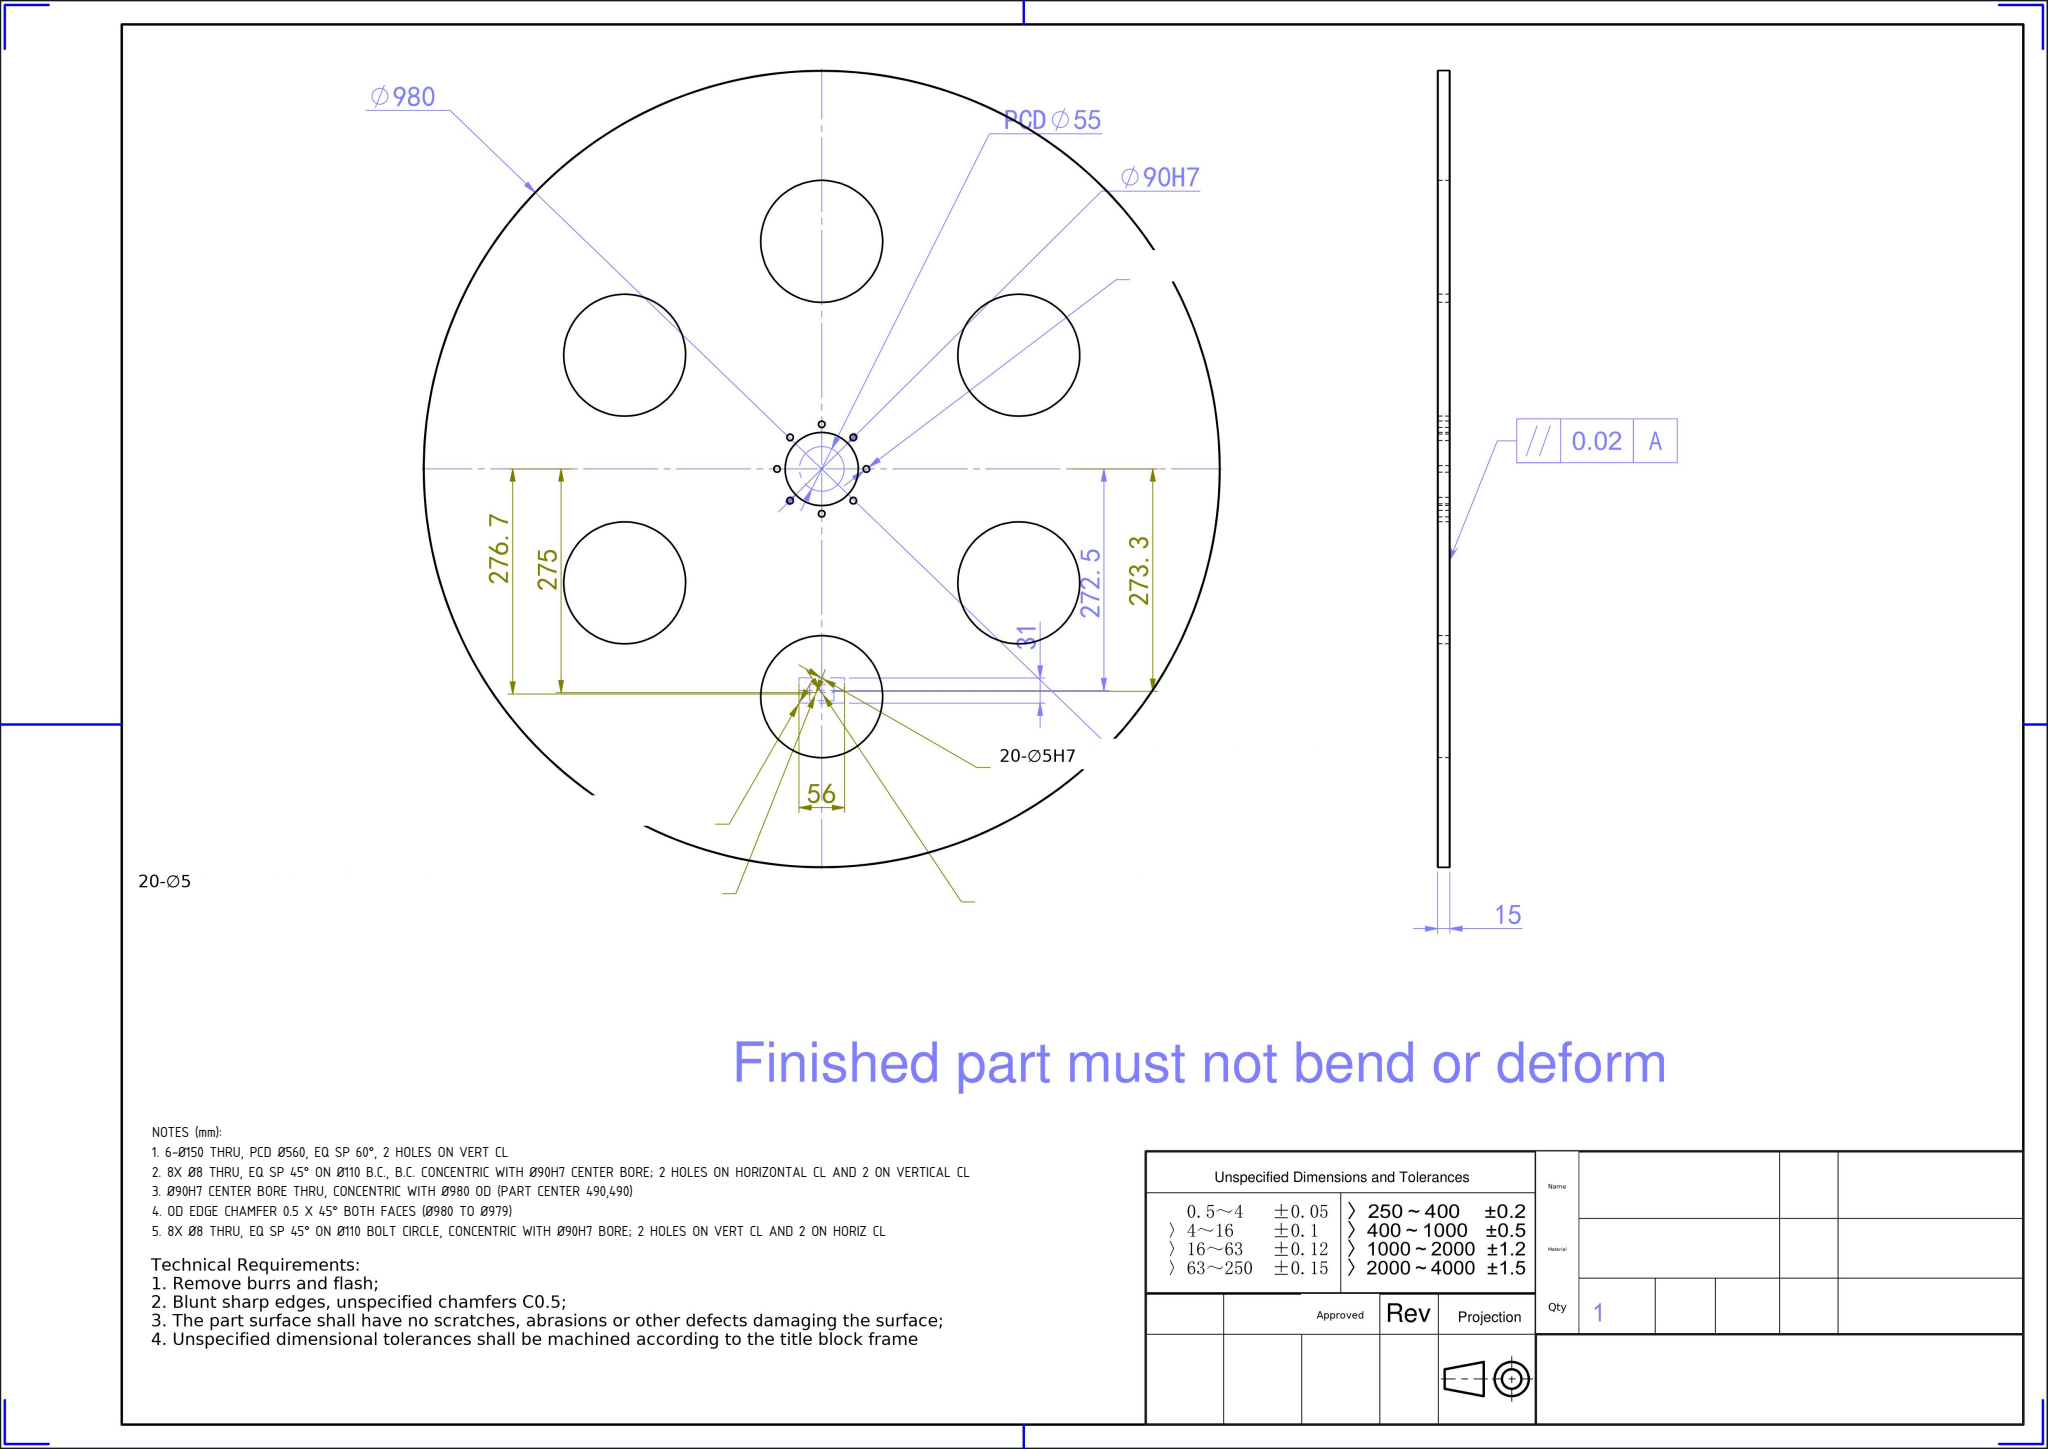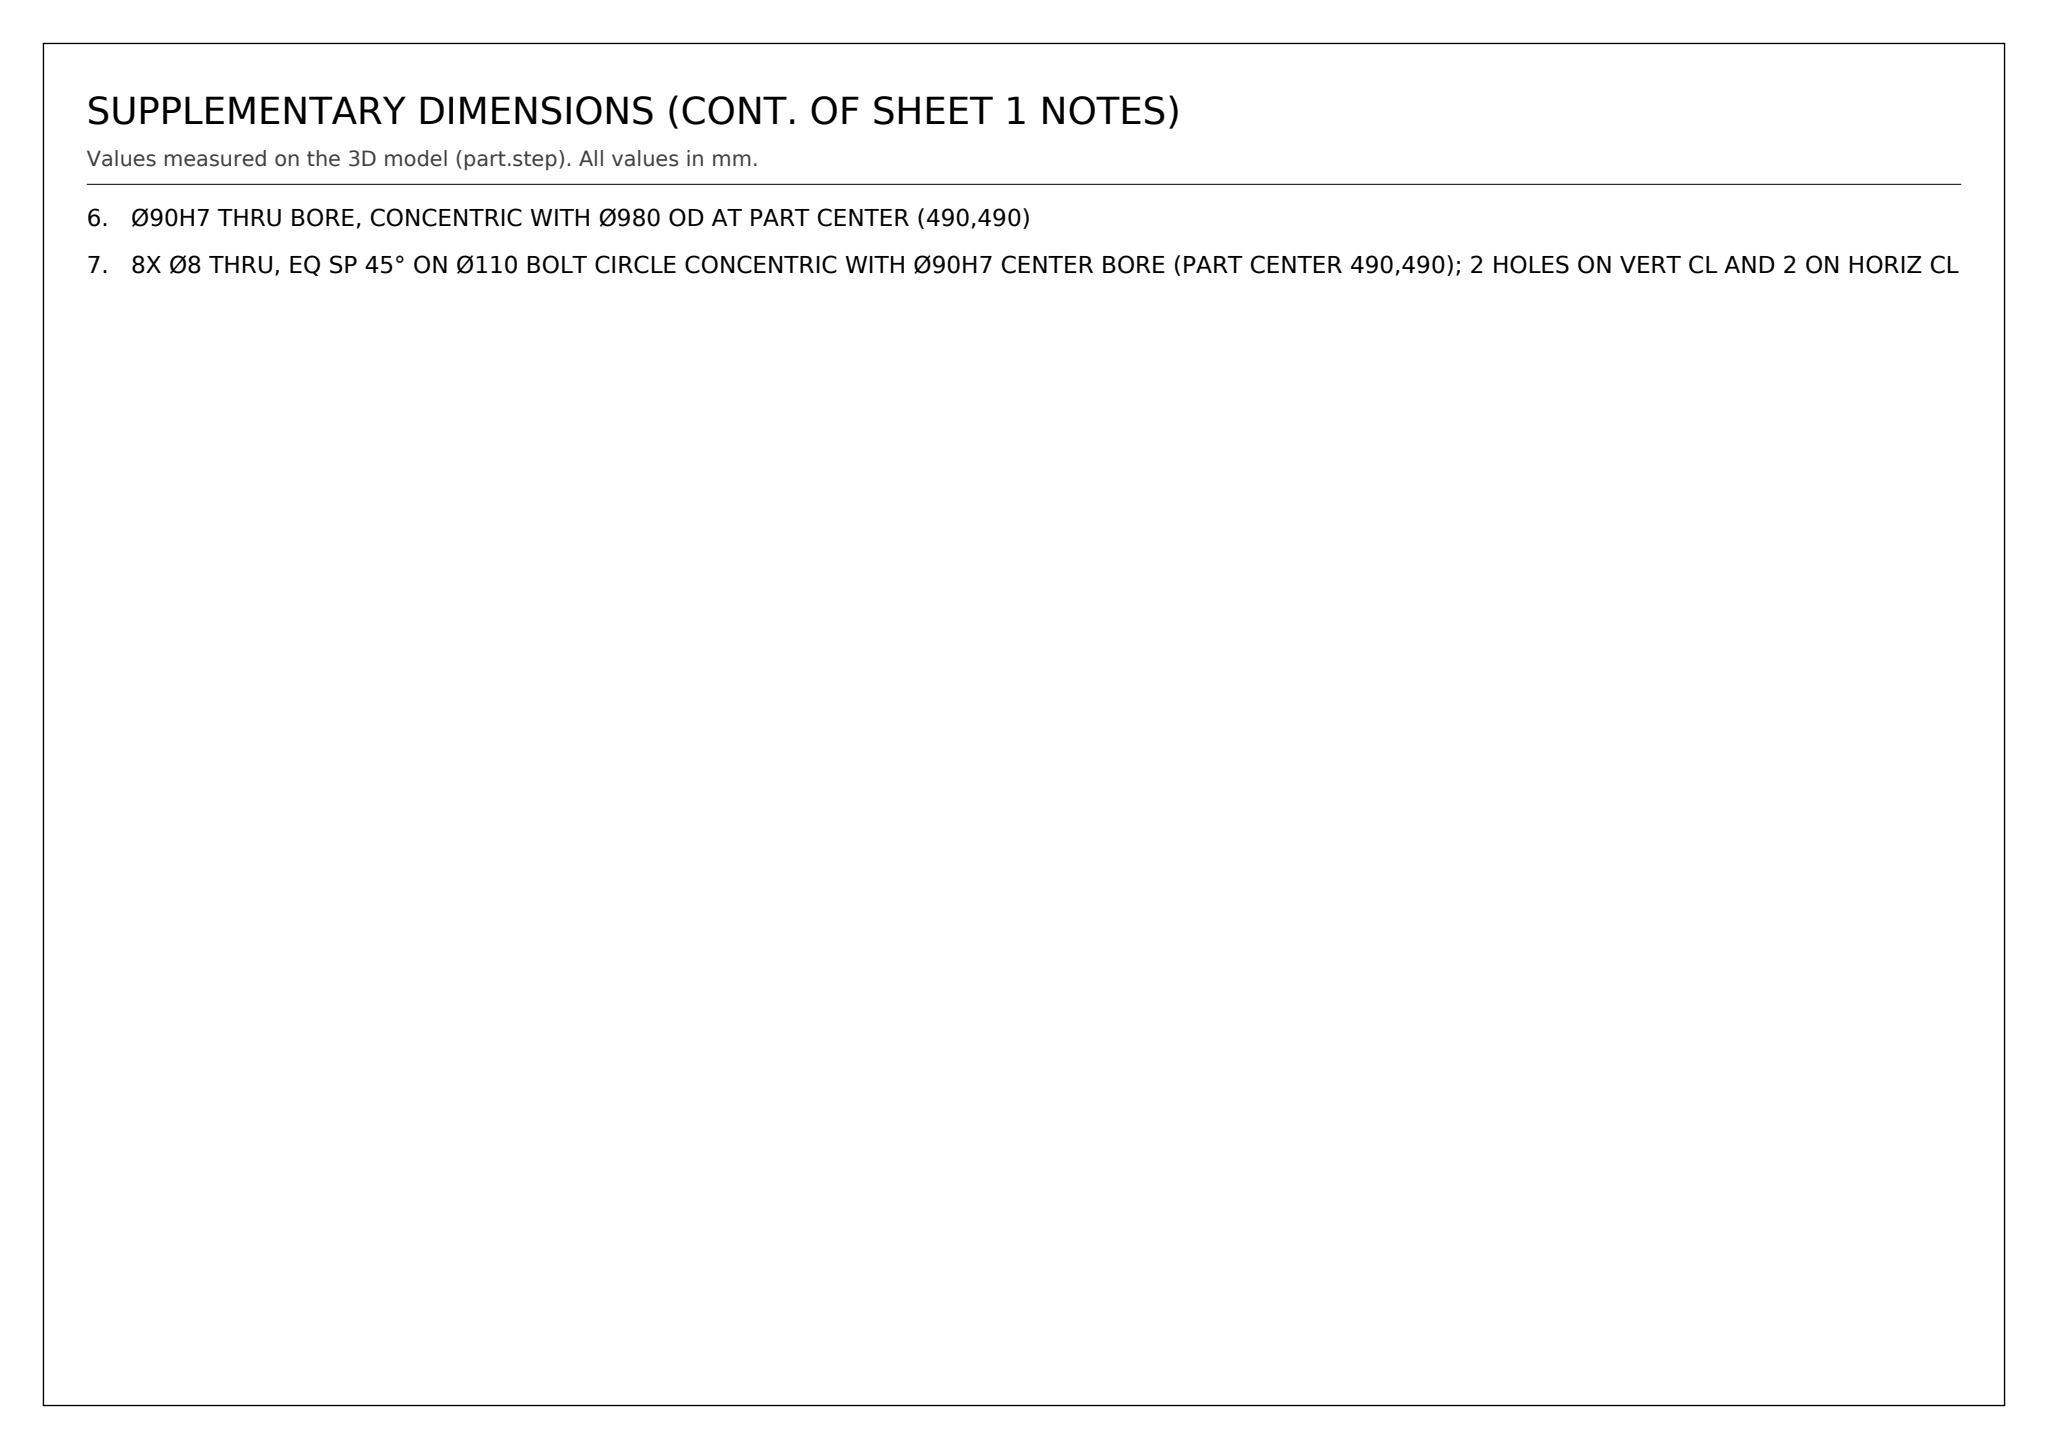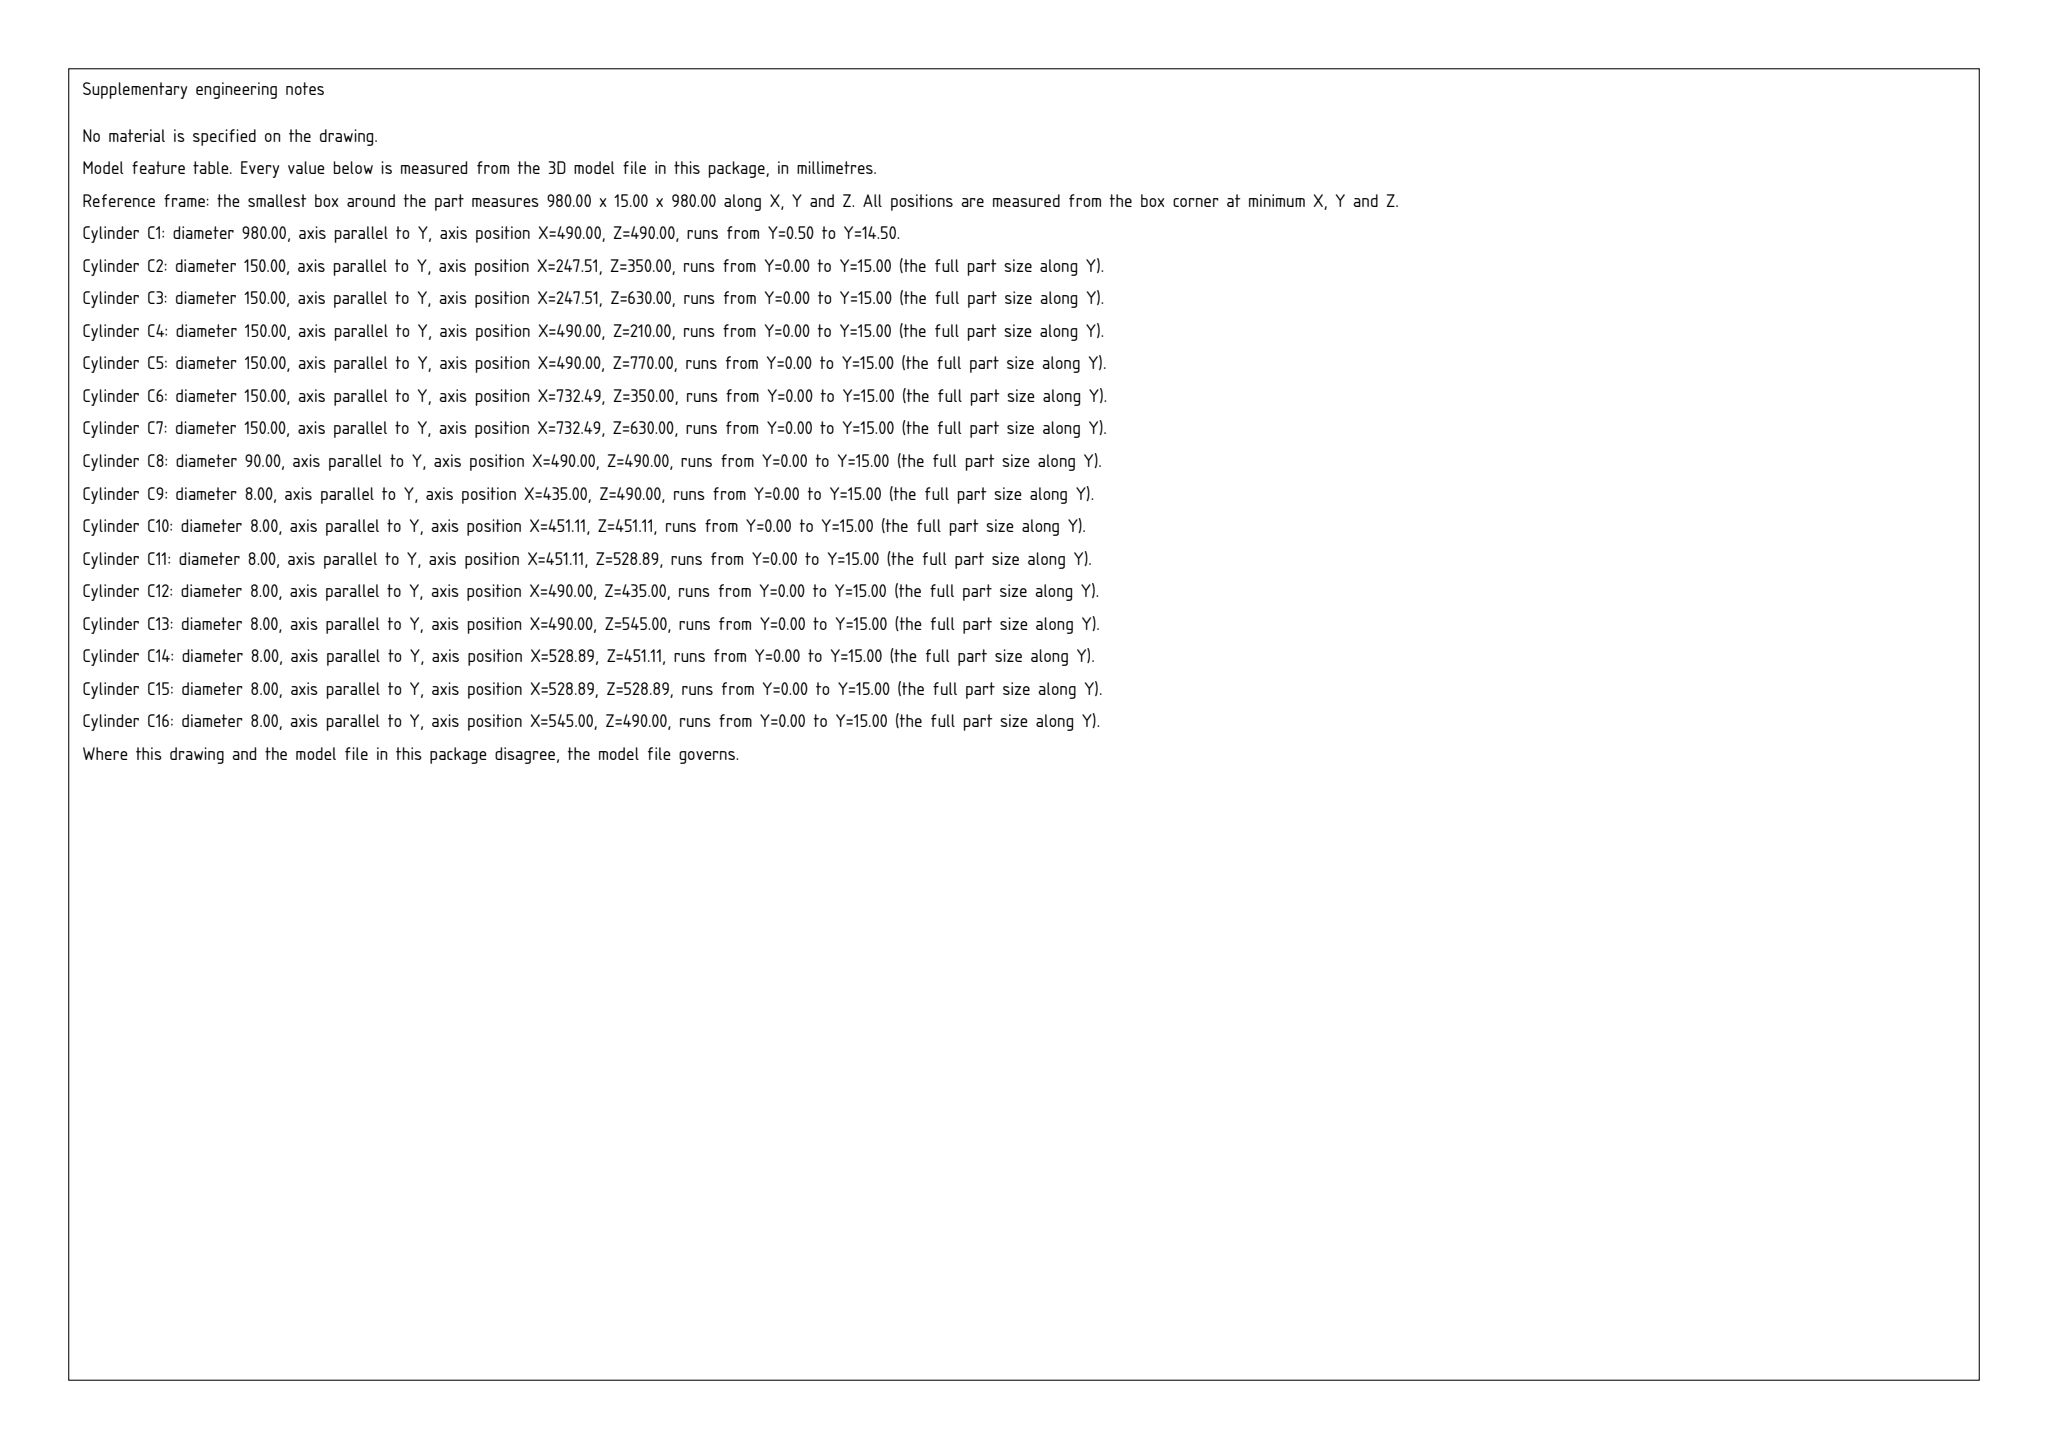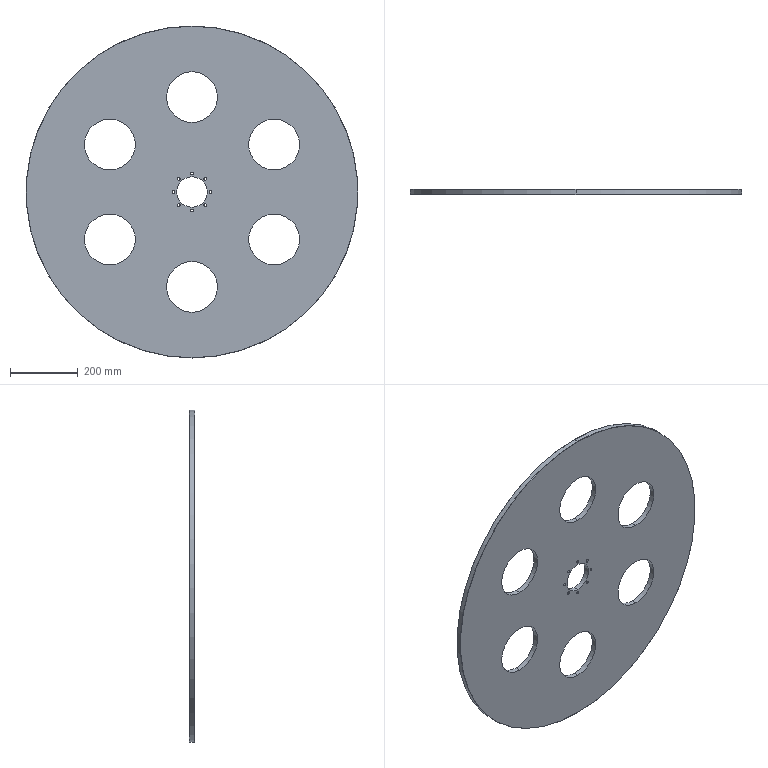Part | SolidWorks | mm | 1 solid | 38 faces | box 980 x 15 x 980 mm | volume 9621787 mm3 | cylinder 32 | cone 4 | plane 2 | commonest cylinder face diameters 8 x16 150 x12 90 x2 980 x2
Drawing notes:
6-Ø150 THRU, PCD Ø560, EQ SP 60°, 2 HOLES ON VERT CL | from the solid: Six Ø150 y-axis cylinders at (247.51,350),(247.51,630),(490,210),(490,770),(732.49,350),(732.49,630); radius from Ø980 centre (490,490) = 280, spacing 60°, two on vertical CL
8X Ø8 THRU, EQ SP 45° ON Ø110 B.C., B.C. CONCENTRIC WITH Ø90H7 CENTER BORE; 2 HOLES ON HORIZONTAL CL AND 2 ON VERTICAL CL | from the solid: cylinders dia 8.0, axis y, 8 positions (435,490),(451.11,451.11),(451.11,528.89),(490,435),(490,545),(528.89,451.11),(528.89,528.89),(545,490) = radius 55 about (490,490)
Ø90H7 CENTER BORE THRU, CONCENTRIC WITH Ø980 OD (PART CENTER 490,490) | from the solid: cylinder dia 90.0, axis y, pos (490,490), length 15; cylinder dia 980.0 at (490,490)
OD EDGE CHAMFER 0.5 X 45° BOTH FACES (Ø980 TO Ø979) | from the solid: cones included angle 90°, ref dia 980.0 and 979.0, 2 each
8X Ø8 THRU, EQ SP 45° ON Ø110 BOLT CIRCLE, CONCENTRIC WITH Ø90H7 BORE; 2 HOLES ON VERT CL AND 2 ON HORIZ CL | from the solid: cylinders dia 8.0, axis y, length 15.0, eight positions (435,490),(451.11,451.11),(451.11,528.89),(490,435),(490,545),(528.89,451.11),(528.89,528.89),(545,490) = R55 about center (490,490)
Ø90H7 THRU BORE, CONCENTRIC WITH Ø980 OD AT PART CENTER (490,490) | from the solid: cylinder dia 90.0, axis y, pos (490,490), length 15.0; cylinder dia 980.0 at pos (490,490)
8X Ø8 THRU, EQ SP 45° ON Ø110 BOLT CIRCLE CONCENTRIC WITH Ø90H7 CENTER BORE (PART CENTER 490,490); 2 HOLES ON VERT CL AND 2 ON HORIZ CL | from the solid: cylinders dia 8.0 axis y at (435,490),(545,490),(490,435),(490,545),(451.11,451.11),(451.11,528.89),(528.89,451.11),(528.89,528.89), length 15 = radius 55 about center (490,490)
build123d program:
from build123d import *

# Parameters (mm, degrees)
SKETCH1_R           = 490
SKETCH1_R_2         = 45
BOSS_EXTRUDE1_DEPTH = 15
CIRPATTERN1_COUNT   = 8
CHAMFER1_SIZE       = 0.5
SKETCH15_R          = 75
CUT_EXTRUDE6_DEPTH  = 20
CIRPATTERN7_COUNT   = 6


with BuildPart() as part:
    # Sketch1 → Boss-Extrude1 (new body)
    with BuildSketch(Plane(origin=(0, 0, 0), x_dir=(1, 0, 0), z_dir=(0, 1, 0))):
        with Locations(Location((0, 0, 0), (0, 0, 270))):
            Circle(SKETCH1_R)
        with Locations(Location((0, 0, 0), (0, 0, 270))):
            Circle(SKETCH1_R_2, mode=Mode.SUBTRACT)
    extrude(amount=BOSS_EXTRUDE1_DEPTH)

    # Sketch3 → 8.0 _8_ Diameter Hole1 (revolve, cut)
    with BuildSketch(Plane(origin=(38.891, 15, 38.891), x_dir=(0, 0, 1), z_dir=(1, 0, 0))):
        Polygon((0, 0), (0, 37.403), (4, 35), (4, 0), align=None)
    f_8_0_8_diameter_hole1 = revolve(axis=Axis((38.891, 21.35, 38.891), (0, -1, 0)), mode=Mode.SUBTRACT)

    # CirPattern1: 8.0 _8_ Diameter Hole1 ×8 about axis
    cirpattern1_axis = Axis((0, 0, 0), (0, 1, 0))
    for i in range(1, CIRPATTERN1_COUNT):
        add(f_8_0_8_diameter_hole1.rotate(cirpattern1_axis, i * 360 / CIRPATTERN1_COUNT), mode=Mode.SUBTRACT)

    # Chamfer1
    chamfer1_edges = [part.edges().sort_by_distance(p)[0] for p in [
        (0, 0, -490),
        (0, 15, -490),
    ]]
    chamfer(chamfer1_edges, length=CHAMFER1_SIZE)

    # Sketch15 → Cut-Extrude6 (cut)
    with BuildSketch(Plane(origin=(0, 15, 0), x_dir=(1, 0, 0), z_dir=(0, 1, 0))):
        with Locations(Location((0, 280, 0), (0, 0, 270))):
            Circle(SKETCH15_R)
    cut_extrude6 = extrude(amount=-CUT_EXTRUDE6_DEPTH, mode=Mode.SUBTRACT)

    # CirPattern7: Cut-Extrude6 ×6 about axis
    cirpattern7_axis = Axis((0, 0, 0), (0, 1, 0))
    for i in range(1, CIRPATTERN7_COUNT):
        add(cut_extrude6.rotate(cirpattern7_axis, i * 360 / CIRPATTERN7_COUNT), mode=Mode.SUBTRACT)


solid = part.part